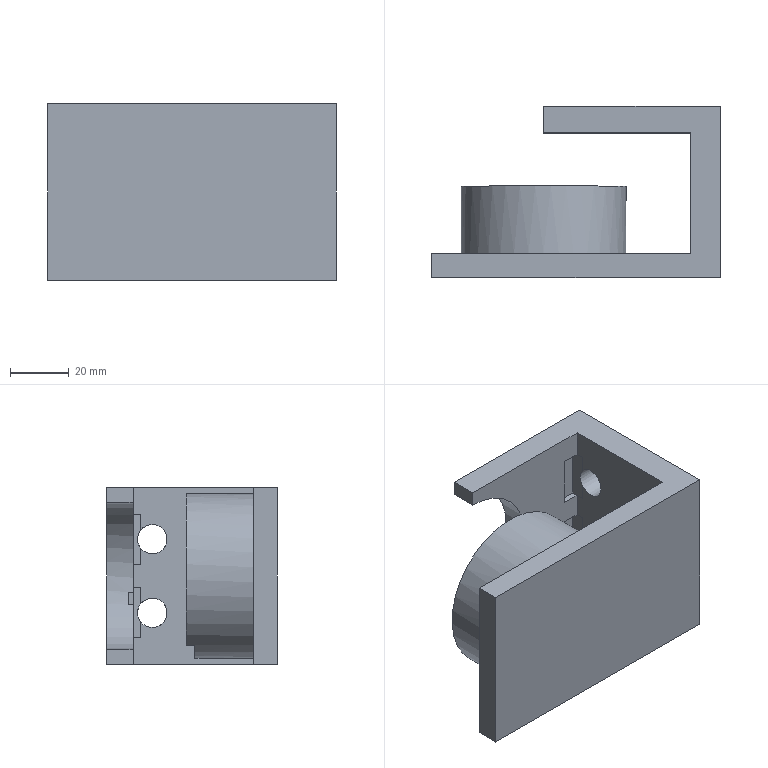Component | NX | DRILL_BUSH_ACC | 1 solid | 42 faces | volume 142155 mm3 | plane 35 | cylinder 7 | commonest cylinder face diameters 10 x4 50 x2 56 x1